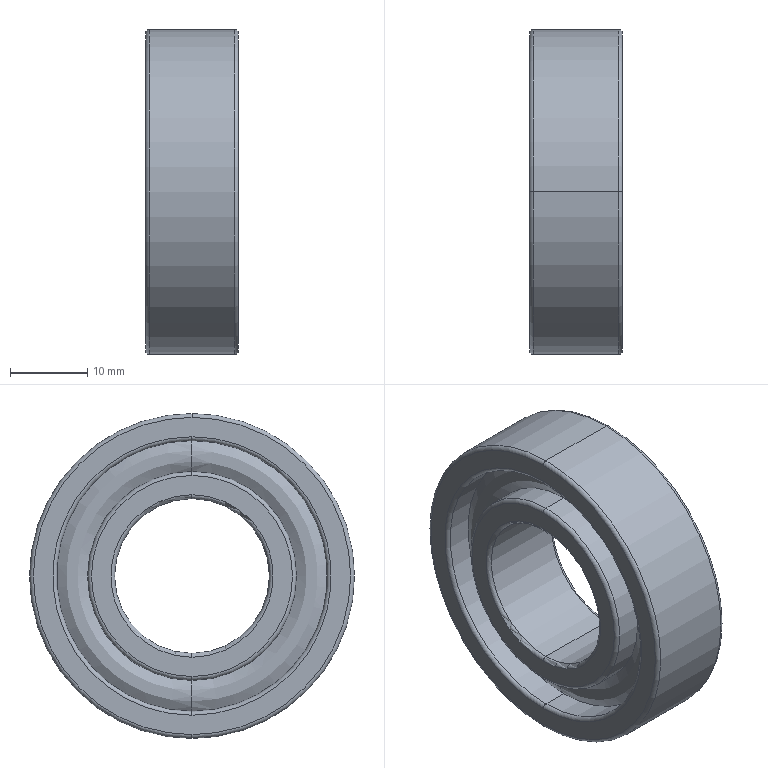Component | SolidWorks | GB-T276  6004RZ-2 | 1 solid | 36 faces | box 12 x 42 x 42 mm | volume 10289 mm3 | torus 20 | cylinder 12 | plane 4 | commonest cylinder face diameters 27 x4 35 x4 42 x2 20 x2 | material '-
build123d program:
from build123d import *

# Parameters (mm, degrees)
FILLET1_R = 0.5


with BuildPart() as part:
    # Sketch1 → Revolve1 (revolve)
    with BuildSketch(Plane.XY, mode=Mode.PRIVATE) as revolve1_sk:
        with BuildLine():
            Line((0, 10), (12, 10))
            Line((12, 10), (12, 13.5))
            Line((12, 13.5), (8.236, 13.5))
            ThreePointArc((8.236, 13.5), (9, 15.5), (8.236, 17.5))
            Line((8.236, 17.5), (12, 17.5))
            Line((12, 17.5), (12, 21))
            Line((12, 21), (0, 21))
            Line((0, 21), (0, 17.5))
            Line((0, 17.5), (3.764, 17.5))
            ThreePointArc((3.764, 17.5), (3, 15.5), (3.764, 13.5))
            Line((3.764, 13.5), (0, 13.5))
            Line((0, 13.5), (0, 10))
        make_face()
    revolve(revolve1_sk.sketch.rotate(Axis((0, 0, 0), (1, 0, 0)), 90), axis=Axis((0, 0, 0), (1, 0, 0)))

    # Fillet1
    fillet1_edges = [part.edges().sort_by_distance(p)[0] for p in [
        (0, 0, -21),
        (12, 0, -21),
        (12, 0, -17.5),
        (12, 0, -13.5),
        (12, 0, -10),
        (0, 0, -10),
        (0, 0, -13.5),
        (0, 0, -17.5),
    ]]
    fillet(fillet1_edges, radius=FILLET1_R)


solid = part.part

# Placed as in the assembly
solid = solid.moved(Location((477, 30, 0), (0, 0, 0)))
STEP:
#1=CARTESIAN_POINT('',(18.78,1.181,-0.5118));
#2=VERTEX_POINT('',#1);
#3=CARTESIAN_POINT('',(18.78,1.181,0.5118));
#4=VERTEX_POINT('',#3);
#5=CARTESIAN_POINT('',(18.78,1.181,-0.));
#6=DIRECTION('',(-1.,-0.,0.));
#7=DIRECTION('',(0.,-0.,1.));
#8=AXIS2_PLACEMENT_3D('',#5,#6,#7);
#9=CIRCLE('',#8,0.5118);
#10=EDGE_CURVE('',#2,#4,#9,.T.);
#11=ORIENTED_EDGE('',*,*,#10,.F.);
#12=CARTESIAN_POINT('',(18.799,1.181,-0.5315));
#13=VERTEX_POINT('',#12);
#14=CARTESIAN_POINT('',(18.799,1.181,-0.5118));
#15=DIRECTION('',(0.,-1.,-0.));
#16=DIRECTION('',(0.,0.,-1.));
#17=AXIS2_PLACEMENT_3D('',#14,#15,#16);
#18=CIRCLE('',#17,0.01969);
#19=EDGE_CURVE('',#2,#13,#18,.T.);
#20=ORIENTED_EDGE('',*,*,#19,.T.);
#21=CARTESIAN_POINT('',(18.799,1.181,0.5315));
#22=VERTEX_POINT('',#21);
#23=CARTESIAN_POINT('',(18.799,1.181,-0.));
#24=DIRECTION('',(1.,0.,-0.));
#25=DIRECTION('',(0.,-0.,1.));
#26=AXIS2_PLACEMENT_3D('',#23,#24,#25);
#27=CIRCLE('',#26,0.5315);
#28=EDGE_CURVE('',#22,#13,#27,.T.);
#29=ORIENTED_EDGE('',*,*,#28,.F.);
#30=CARTESIAN_POINT('',(18.799,1.181,0.5118));
#31=DIRECTION('',(-0.,1.,0.));
#32=DIRECTION('',(0.,0.,1.));
#33=AXIS2_PLACEMENT_3D('',#30,#31,#32);
#34=CIRCLE('',#33,0.01969);
#35=EDGE_CURVE('',#4,#22,#34,.T.);
#36=ORIENTED_EDGE('',*,*,#35,.F.);
#37=EDGE_LOOP('',(#11,#20,#29,#36));
#38=FACE_OUTER_BOUND('',#37,.T.);
#39=CARTESIAN_POINT('',(18.799,1.181,-0.));
#40=DIRECTION('',(1.,0.,-0.));
#41=DIRECTION('',(0.,-0.,1.));
#42=AXIS2_PLACEMENT_3D('',#39,#40,#41);
#43=TOROIDAL_SURFACE('',#42,0.5118,0.01969);
#44=ADVANCED_FACE('',(#38),#43,.T.);
#45=CARTESIAN_POINT('',(18.799,1.181,-0.3937));
#46=VERTEX_POINT('',#45);
#47=CARTESIAN_POINT('',(18.799,1.181,0.3937));
#48=VERTEX_POINT('',#47);
#49=CARTESIAN_POINT('',(18.799,1.181,-0.));
#50=DIRECTION('',(-1.,-0.,0.));
#51=DIRECTION('',(0.,-0.,1.));
#52=AXIS2_PLACEMENT_3D('',#49,#50,#51);
#53=CIRCLE('',#52,0.3937);
#54=EDGE_CURVE('',#46,#48,#53,.T.);
#55=ORIENTED_EDGE('',*,*,#54,.F.);
#56=CARTESIAN_POINT('',(18.78,1.181,-0.4134));
#57=VERTEX_POINT('',#56);
#58=CARTESIAN_POINT('',(18.799,1.181,-0.4134));
#59=DIRECTION('',(0.,-1.,-0.));
#60=DIRECTION('',(0.,0.,-1.));
#61=AXIS2_PLACEMENT_3D('',#58,#59,#60);
#62=CIRCLE('',#61,0.01969);
#63=EDGE_CURVE('',#46,#57,#62,.T.);
#64=ORIENTED_EDGE('',*,*,#63,.T.);
#65=CARTESIAN_POINT('',(18.78,1.181,0.4134));
#66=VERTEX_POINT('',#65);
#67=CARTESIAN_POINT('',(18.78,1.181,-0.));
#68=DIRECTION('',(1.,0.,-0.));
#69=DIRECTION('',(0.,-0.,1.));
#70=AXIS2_PLACEMENT_3D('',#67,#68,#69);
#71=CIRCLE('',#70,0.4134);
#72=EDGE_CURVE('',#66,#57,#71,.T.);
#73=ORIENTED_EDGE('',*,*,#72,.F.);
#74=CARTESIAN_POINT('',(18.799,1.181,0.4134));
#75=DIRECTION('',(-0.,1.,0.));
#76=DIRECTION('',(0.,0.,1.));
#77=AXIS2_PLACEMENT_3D('',#74,#75,#76);
#78=CIRCLE('',#77,0.01969);
#79=EDGE_CURVE('',#48,#66,#78,.T.);
#80=ORIENTED_EDGE('',*,*,#79,.F.);
#81=EDGE_LOOP('',(#55,#64,#73,#80));
#82=FACE_OUTER_BOUND('',#81,.T.);
#83=CARTESIAN_POINT('',(18.799,1.181,-0.));
#84=DIRECTION('',(1.,0.,-0.));
#85=DIRECTION('',(0.,-0.,1.));
#86=AXIS2_PLACEMENT_3D('',#83,#84,#85);
#87=TOROIDAL_SURFACE('',#86,0.4134,0.01969);
#88=ADVANCED_FACE('',(#82),#87,.T.);
#89=CARTESIAN_POINT('',(18.78,1.181,-0.8071));
#90=VERTEX_POINT('',#89);
#91=CARTESIAN_POINT('',(18.78,1.181,0.8071));
#92=VERTEX_POINT('',#91);
#93=CARTESIAN_POINT('',(18.78,1.181,-0.));
#94=DIRECTION('',(-1.,-0.,0.));
#95=DIRECTION('',(0.,-0.,1.));
#96=AXIS2_PLACEMENT_3D('',#93,#94,#95);
#97=CIRCLE('',#96,0.8071);
#98=EDGE_CURVE('',#90,#92,#97,.T.);
#99=ORIENTED_EDGE('',*,*,#98,.F.);
#100=CARTESIAN_POINT('',(18.799,1.181,-0.8268));
#101=VERTEX_POINT('',#100);
#102=CARTESIAN_POINT('',(18.799,1.181,-0.8071));
#103=DIRECTION('',(0.,-1.,-0.));
#104=DIRECTION('',(0.,0.,-1.));
#105=AXIS2_PLACEMENT_3D('',#102,#103,#104);
#106=CIRCLE('',#105,0.01969);
#107=EDGE_CURVE('',#90,#101,#106,.T.);
#108=ORIENTED_EDGE('',*,*,#107,.T.);
#109=CARTESIAN_POINT('',(18.799,1.181,0.8268));
#110=VERTEX_POINT('',#109);
#111=CARTESIAN_POINT('',(18.799,1.181,-0.));
#112=DIRECTION('',(1.,0.,-0.));
#113=DIRECTION('',(0.,-0.,1.));
#114=AXIS2_PLACEMENT_3D('',#111,#112,#113);
#115=CIRCLE('',#114,0.8268);
#116=EDGE_CURVE('',#110,#101,#115,.T.);
#117=ORIENTED_EDGE('',*,*,#116,.F.);
#118=CARTESIAN_POINT('',(18.799,1.181,0.8071));
#119=DIRECTION('',(-0.,1.,0.));
#120=DIRECTION('',(0.,0.,1.));
#121=AXIS2_PLACEMENT_3D('',#118,#119,#120);
#122=CIRCLE('',#121,0.01969);
#123=EDGE_CURVE('',#92,#110,#122,.T.);
#124=ORIENTED_EDGE('',*,*,#123,.F.);
#125=EDGE_LOOP('',(#99,#108,#117,#124));
#126=FACE_OUTER_BOUND('',#125,.T.);
#127=CARTESIAN_POINT('',(18.799,1.181,-0.));
#128=DIRECTION('',(1.,0.,-0.));
#129=DIRECTION('',(0.,-0.,1.));
#130=AXIS2_PLACEMENT_3D('',#127,#128,#129);
#131=TOROIDAL_SURFACE('',#130,0.8071,0.01969);
#132=ADVANCED_FACE('',(#126),#131,.T.);
#133=CARTESIAN_POINT('',(18.799,1.181,-0.689));
#134=VERTEX_POINT('',#133);
#135=CARTESIAN_POINT('',(18.799,1.181,0.689));
#136=VERTEX_POINT('',#135);
#137=CARTESIAN_POINT('',(18.799,1.181,-0.));
#138=DIRECTION('',(-1.,-0.,0.));
#139=DIRECTION('',(0.,-0.,1.));
#140=AXIS2_PLACEMENT_3D('',#137,#138,#139);
#141=CIRCLE('',#140,0.689);
#142=EDGE_CURVE('',#134,#136,#141,.T.);
#143=ORIENTED_EDGE('',*,*,#142,.F.);
#144=CARTESIAN_POINT('',(18.78,1.181,-0.7087));
#145=VERTEX_POINT('',#144);
#146=CARTESIAN_POINT('',(18.799,1.181,-0.7087));
#147=DIRECTION('',(0.,-1.,-0.));
#148=DIRECTION('',(0.,0.,-1.));
#149=AXIS2_PLACEMENT_3D('',#146,#147,#148);
#150=CIRCLE('',#149,0.01969);
#151=EDGE_CURVE('',#134,#145,#150,.T.);
#152=ORIENTED_EDGE('',*,*,#151,.T.);
#153=CARTESIAN_POINT('',(18.78,1.181,0.7087));
#154=VERTEX_POINT('',#153);
#155=CARTESIAN_POINT('',(18.78,1.181,-0.));
#156=DIRECTION('',(1.,0.,-0.));
#157=DIRECTION('',(0.,-0.,1.));
#158=AXIS2_PLACEMENT_3D('',#155,#156,#157);
#159=CIRCLE('',#158,0.7087);
#160=EDGE_CURVE('',#154,#145,#159,.T.);
#161=ORIENTED_EDGE('',*,*,#160,.F.);
#162=CARTESIAN_POINT('',(18.799,1.181,0.7087));
#163=DIRECTION('',(-0.,1.,0.));
#164=DIRECTION('',(0.,0.,1.));
#165=AXIS2_PLACEMENT_3D('',#162,#163,#164);
#166=CIRCLE('',#165,0.01969);
#167=EDGE_CURVE('',#136,#154,#166,.T.);
#168=ORIENTED_EDGE('',*,*,#167,.F.);
#169=EDGE_LOOP('',(#143,#152,#161,#168));
#170=FACE_OUTER_BOUND('',#169,.T.);
#171=CARTESIAN_POINT('',(18.799,1.181,-0.));
#172=DIRECTION('',(1.,0.,-0.));
#173=DIRECTION('',(0.,-0.,1.));
#174=AXIS2_PLACEMENT_3D('',#171,#172,#173);
#175=TOROIDAL_SURFACE('',#174,0.7087,0.01969);
#176=ADVANCED_FACE('',(#170),#175,.T.);
#177=CARTESIAN_POINT('',(19.232,1.181,0.3937));
#178=VERTEX_POINT('',#177);
#179=CARTESIAN_POINT('',(19.232,1.181,-0.3937));
#180=VERTEX_POINT('',#179);
#181=CARTESIAN_POINT('',(19.232,1.181,-0.));
#182=DIRECTION('',(1.,0.,-0.));
#183=DIRECTION('',(0.,0.,-1.));
#184=AXIS2_PLACEMENT_3D('',#181,#182,#183);
#185=CIRCLE('',#184,0.3937);
#186=EDGE_CURVE('',#178,#180,#185,.T.);
#187=ORIENTED_EDGE('',*,*,#186,.F.);
#188=CARTESIAN_POINT('',(19.252,1.181,0.4134));
#189=VERTEX_POINT('',#188);
#190=CARTESIAN_POINT('',(19.232,1.181,0.4134));
#191=DIRECTION('',(0.,-1.,-0.));
#192=DIRECTION('',(0.,0.,-1.));
#193=AXIS2_PLACEMENT_3D('',#190,#191,#192);
#194=CIRCLE('',#193,0.01969);
#195=EDGE_CURVE('',#178,#189,#194,.T.);
#196=ORIENTED_EDGE('',*,*,#195,.T.);
#197=CARTESIAN_POINT('',(19.252,1.181,-0.4134));
#198=VERTEX_POINT('',#197);
#199=CARTESIAN_POINT('',(19.252,1.181,-0.));
#200=DIRECTION('',(-1.,-0.,0.));
#201=DIRECTION('',(0.,0.,-1.));
#202=AXIS2_PLACEMENT_3D('',#199,#200,#201);
#203=CIRCLE('',#202,0.4134);
#204=EDGE_CURVE('',#198,#189,#203,.T.);
#205=ORIENTED_EDGE('',*,*,#204,.F.);
#206=CARTESIAN_POINT('',(19.232,1.181,-0.4134));
#207=DIRECTION('',(-0.,1.,0.));
#208=DIRECTION('',(0.,0.,1.));
#209=AXIS2_PLACEMENT_3D('',#206,#207,#208);
#210=CIRCLE('',#209,0.01969);
#211=EDGE_CURVE('',#180,#198,#210,.T.);
#212=ORIENTED_EDGE('',*,*,#211,.F.);
#213=EDGE_LOOP('',(#187,#196,#205,#212));
#214=FACE_OUTER_BOUND('',#213,.T.);
#215=CARTESIAN_POINT('',(19.232,1.181,-0.));
#216=DIRECTION('',(-1.,-0.,0.));
#217=DIRECTION('',(-0.,0.,-1.));
#218=AXIS2_PLACEMENT_3D('',#215,#216,#217);
#219=TOROIDAL_SURFACE('',#218,0.4134,0.01969);
#220=ADVANCED_FACE('',(#214),#219,.T.);
#221=CARTESIAN_POINT('',(19.252,1.181,0.5118));
#222=VERTEX_POINT('',#221);
#223=CARTESIAN_POINT('',(19.252,1.181,-0.5118));
#224=VERTEX_POINT('',#223);
#225=CARTESIAN_POINT('',(19.252,1.181,-0.));
#226=DIRECTION('',(1.,0.,-0.));
#227=DIRECTION('',(0.,0.,-1.));
#228=AXIS2_PLACEMENT_3D('',#225,#226,#227);
#229=CIRCLE('',#228,0.5118);
#230=EDGE_CURVE('',#222,#224,#229,.T.);
#231=ORIENTED_EDGE('',*,*,#230,.F.);
#232=CARTESIAN_POINT('',(19.232,1.181,0.5315));
#233=VERTEX_POINT('',#232);
#234=CARTESIAN_POINT('',(19.232,1.181,0.5118));
#235=DIRECTION('',(0.,-1.,-0.));
#236=DIRECTION('',(0.,0.,-1.));
#237=AXIS2_PLACEMENT_3D('',#234,#235,#236);
#238=CIRCLE('',#237,0.01969);
#239=EDGE_CURVE('',#222,#233,#238,.T.);
#240=ORIENTED_EDGE('',*,*,#239,.T.);
#241=CARTESIAN_POINT('',(19.232,1.181,-0.5315));
#242=VERTEX_POINT('',#241);
#243=CARTESIAN_POINT('',(19.232,1.181,-0.));
#244=DIRECTION('',(-1.,-0.,0.));
#245=DIRECTION('',(0.,0.,-1.));
#246=AXIS2_PLACEMENT_3D('',#243,#244,#245);
#247=CIRCLE('',#246,0.5315);
#248=EDGE_CURVE('',#242,#233,#247,.T.);
#249=ORIENTED_EDGE('',*,*,#248,.F.);
#250=CARTESIAN_POINT('',(19.232,1.181,-0.5118));
#251=DIRECTION('',(-0.,1.,0.));
#252=DIRECTION('',(0.,0.,1.));
#253=AXIS2_PLACEMENT_3D('',#250,#251,#252);
#254=CIRCLE('',#253,0.01969);
#255=EDGE_CURVE('',#224,#242,#254,.T.);
#256=ORIENTED_EDGE('',*,*,#255,.F.);
#257=EDGE_LOOP('',(#231,#240,#249,#256));
#258=FACE_OUTER_BOUND('',#257,.T.);
#259=CARTESIAN_POINT('',(19.232,1.181,-0.));
#260=DIRECTION('',(-1.,-0.,0.));
#261=DIRECTION('',(-0.,0.,-1.));
#262=AXIS2_PLACEMENT_3D('',#259,#260,#261);
#263=TOROIDAL_SURFACE('',#262,0.5118,0.01969);
#264=ADVANCED_FACE('',(#258),#263,.T.);
#265=CARTESIAN_POINT('',(19.232,1.181,0.689));
#266=VERTEX_POINT('',#265);
#267=CARTESIAN_POINT('',(19.232,1.181,-0.689));
#268=VERTEX_POINT('',#267);
#269=CARTESIAN_POINT('',(19.232,1.181,-0.));
#270=DIRECTION('',(1.,0.,-0.));
#271=DIRECTION('',(0.,0.,-1.));
#272=AXIS2_PLACEMENT_3D('',#269,#270,#271);
#273=CIRCLE('',#272,0.689);
#274=EDGE_CURVE('',#266,#268,#273,.T.);
#275=ORIENTED_EDGE('',*,*,#274,.F.);
#276=CARTESIAN_POINT('',(19.252,1.181,0.7087));
#277=VERTEX_POINT('',#276);
#278=CARTESIAN_POINT('',(19.232,1.181,0.7087));
#279=DIRECTION('',(0.,-1.,-0.));
#280=DIRECTION('',(0.,0.,-1.));
#281=AXIS2_PLACEMENT_3D('',#278,#279,#280);
#282=CIRCLE('',#281,0.01969);
#283=EDGE_CURVE('',#266,#277,#282,.T.);
#284=ORIENTED_EDGE('',*,*,#283,.T.);
#285=CARTESIAN_POINT('',(19.252,1.181,-0.7087));
#286=VERTEX_POINT('',#285);
#287=CARTESIAN_POINT('',(19.252,1.181,-0.));
#288=DIRECTION('',(-1.,-0.,0.));
#289=DIRECTION('',(0.,0.,-1.));
#290=AXIS2_PLACEMENT_3D('',#287,#288,#289);
#291=CIRCLE('',#290,0.7087);
#292=EDGE_CURVE('',#286,#277,#291,.T.);
#293=ORIENTED_EDGE('',*,*,#292,.F.);
#294=CARTESIAN_POINT('',(19.232,1.181,-0.7087));
#295=DIRECTION('',(-0.,1.,0.));
#296=DIRECTION('',(0.,0.,1.));
#297=AXIS2_PLACEMENT_3D('',#294,#295,#296);
#298=CIRCLE('',#297,0.01969);
#299=EDGE_CURVE('',#268,#286,#298,.T.);
#300=ORIENTED_EDGE('',*,*,#299,.F.);
#301=EDGE_LOOP('',(#275,#284,#293,#300));
#302=FACE_OUTER_BOUND('',#301,.T.);
#303=CARTESIAN_POINT('',(19.232,1.181,-0.));
#304=DIRECTION('',(-1.,-0.,0.));
#305=DIRECTION('',(-0.,0.,-1.));
#306=AXIS2_PLACEMENT_3D('',#303,#304,#305);
#307=TOROIDAL_SURFACE('',#306,0.7087,0.01969);
#308=ADVANCED_FACE('',(#302),#307,.T.);
#309=CARTESIAN_POINT('',(19.252,1.181,0.8071));
#310=VERTEX_POINT('',#309);
#311=CARTESIAN_POINT('',(19.252,1.181,-0.8071));
#312=VERTEX_POINT('',#311);
#313=CARTESIAN_POINT('',(19.252,1.181,-0.));
#314=DIRECTION('',(1.,0.,-0.));
#315=DIRECTION('',(0.,0.,-1.));
#316=AXIS2_PLACEMENT_3D('',#313,#314,#315);
#317=CIRCLE('',#316,0.8071);
#318=EDGE_CURVE('',#310,#312,#317,.T.);
#319=ORIENTED_EDGE('',*,*,#318,.F.);
#320=CARTESIAN_POINT('',(19.232,1.181,0.8268));
#321=VERTEX_POINT('',#320);
#322=CARTESIAN_POINT('',(19.232,1.181,0.8071));
#323=DIRECTION('',(0.,-1.,-0.));
#324=DIRECTION('',(0.,0.,-1.));
#325=AXIS2_PLACEMENT_3D('',#322,#323,#324);
#326=CIRCLE('',#325,0.01969);
#327=EDGE_CURVE('',#310,#321,#326,.T.);
#328=ORIENTED_EDGE('',*,*,#327,.T.);
#329=CARTESIAN_POINT('',(19.232,1.181,-0.8268));
#330=VERTEX_POINT('',#329);
#331=CARTESIAN_POINT('',(19.232,1.181,-0.));
#332=DIRECTION('',(-1.,-0.,0.));
#333=DIRECTION('',(0.,0.,-1.));
#334=AXIS2_PLACEMENT_3D('',#331,#332,#333);
#335=CIRCLE('',#334,0.8268);
#336=EDGE_CURVE('',#330,#321,#335,.T.);
#337=ORIENTED_EDGE('',*,*,#336,.F.);
#338=CARTESIAN_POINT('',(19.232,1.181,-0.8071));
#339=DIRECTION('',(-0.,1.,0.));
#340=DIRECTION('',(0.,0.,1.));
#341=AXIS2_PLACEMENT_3D('',#338,#339,#340);
#342=CIRCLE('',#341,0.01969);
#343=EDGE_CURVE('',#312,#330,#342,.T.);
#344=ORIENTED_EDGE('',*,*,#343,.F.);
#345=EDGE_LOOP('',(#319,#328,#337,#344));
#346=FACE_OUTER_BOUND('',#345,.T.);
#347=CARTESIAN_POINT('',(19.232,1.181,-0.));
#348=DIRECTION('',(-1.,-0.,0.));
#349=DIRECTION('',(-0.,0.,-1.));
#350=AXIS2_PLACEMENT_3D('',#347,#348,#349);
#351=TOROIDAL_SURFACE('',#350,0.8071,0.01969);
#352=ADVANCED_FACE('',(#346),#351,.T.);
#353=CARTESIAN_POINT('',(19.104,1.181,0.5315));
#354=VERTEX_POINT('',#353);
#355=CARTESIAN_POINT('',(19.104,1.181,-0.5315));
#356=VERTEX_POINT('',#355);
#357=CARTESIAN_POINT('',(19.104,1.181,-0.));
#358=DIRECTION('',(1.,0.,-0.));
#359=DIRECTION('',(0.,-0.,1.));
#360=AXIS2_PLACEMENT_3D('',#357,#358,#359);
#361=CIRCLE('',#360,0.5315);
#362=EDGE_CURVE('',#354,#356,#361,.T.);
#363=ORIENTED_EDGE('',*,*,#362,.T.);
#364=CARTESIAN_POINT('',(19.252,1.181,-0.5315));
#365=DIRECTION('',(1.,0.,-0.));
#366=VECTOR('',#365,39.37);
#367=LINE('',#364,#366);
#368=EDGE_CURVE('',#356,#242,#367,.T.);
#369=ORIENTED_EDGE('',*,*,#368,.T.);
#370=ORIENTED_EDGE('',*,*,#248,.T.);
#371=CARTESIAN_POINT('',(19.252,1.181,0.5315));
#372=DIRECTION('',(1.,0.,-0.));
#373=VECTOR('',#372,39.37);
#374=LINE('',#371,#373);
#375=EDGE_CURVE('',#354,#233,#374,.T.);
#376=ORIENTED_EDGE('',*,*,#375,.F.);
#377=EDGE_LOOP('',(#363,#369,#370,#376));
#378=FACE_OUTER_BOUND('',#377,.T.);
#379=CARTESIAN_POINT('',(19.252,1.181,-0.));
#380=DIRECTION('',(1.,0.,-0.));
#381=DIRECTION('',(0.,-0.,1.));
#382=AXIS2_PLACEMENT_3D('',#379,#380,#381);
#383=CYLINDRICAL_SURFACE('',#382,0.5315);
#384=ADVANCED_FACE('',(#378),#383,.T.);
#385=CARTESIAN_POINT('',(19.104,1.181,0.689));
#386=VERTEX_POINT('',#385);
#387=CARTESIAN_POINT('',(19.104,1.181,-0.689));
#388=VERTEX_POINT('',#387);
#389=CARTESIAN_POINT('',(19.104,1.181,-0.));
#390=DIRECTION('',(1.,0.,-0.));
#391=DIRECTION('',(0.,-0.,1.));
#392=AXIS2_PLACEMENT_3D('',#389,#390,#391);
#393=CIRCLE('',#392,0.689);
#394=EDGE_CURVE('',#386,#388,#393,.T.);
#395=ORIENTED_EDGE('',*,*,#394,.T.);
#396=CARTESIAN_POINT('',(19.016,1.181,-0.6102));
#397=DIRECTION('',(0.,-1.,-0.));
#398=DIRECTION('',(0.,0.,-1.));
#399=AXIS2_PLACEMENT_3D('',#396,#397,#398);
#400=CIRCLE('',#399,0.1181);
#401=EDGE_CURVE('',#388,#356,#400,.T.);
#402=ORIENTED_EDGE('',*,*,#401,.T.);
#403=ORIENTED_EDGE('',*,*,#362,.F.);
#404=CARTESIAN_POINT('',(19.016,1.181,0.6102));
#405=DIRECTION('',(-0.,1.,0.));
#406=DIRECTION('',(0.,0.,1.));
#407=AXIS2_PLACEMENT_3D('',#404,#405,#406);
#408=CIRCLE('',#407,0.1181);
#409=EDGE_CURVE('',#386,#354,#408,.T.);
#410=ORIENTED_EDGE('',*,*,#409,.F.);
#411=EDGE_LOOP('',(#395,#402,#403,#410));
#412=FACE_OUTER_BOUND('',#411,.T.);
#413=CARTESIAN_POINT('',(19.016,1.181,-0.));
#414=DIRECTION('',(1.,0.,-0.));
#415=DIRECTION('',(0.,-0.,1.));
#416=AXIS2_PLACEMENT_3D('',#413,#414,#415);
#417=TOROIDAL_SURFACE('',#416,0.6102,0.1181);
#418=ADVANCED_FACE('',(#412),#417,.T.);
#419=CARTESIAN_POINT('',(19.104,1.181,-0.));
#420=DIRECTION('',(1.,0.,-0.));
#421=DIRECTION('',(0.,-0.,1.));
#422=AXIS2_PLACEMENT_3D('',#419,#420,#421);
#423=CIRCLE('',#422,0.689);
#424=EDGE_CURVE('',#388,#386,#423,.T.);
#425=ORIENTED_EDGE('',*,*,#424,.F.);
#426=CARTESIAN_POINT('',(19.252,1.181,-0.689));
#427=DIRECTION('',(1.,0.,-0.));
#428=VECTOR('',#427,39.37);
#429=LINE('',#426,#428);
#430=EDGE_CURVE('',#388,#268,#429,.T.);
#431=ORIENTED_EDGE('',*,*,#430,.T.);
#432=CARTESIAN_POINT('',(19.232,1.181,-0.));
#433=DIRECTION('',(1.,0.,-0.));
#434=DIRECTION('',(0.,0.,-1.));
#435=AXIS2_PLACEMENT_3D('',#432,#433,#434);
#436=CIRCLE('',#435,0.689);
#437=EDGE_CURVE('',#268,#266,#436,.T.);
#438=ORIENTED_EDGE('',*,*,#437,.T.);
#439=CARTESIAN_POINT('',(19.252,1.181,0.689));
#440=DIRECTION('',(1.,0.,-0.));
#441=VECTOR('',#440,39.37);
#442=LINE('',#439,#441);
#443=EDGE_CURVE('',#386,#266,#442,.T.);
#444=ORIENTED_EDGE('',*,*,#443,.F.);
#445=EDGE_LOOP('',(#425,#431,#438,#444));
#446=FACE_OUTER_BOUND('',#445,.T.);
#447=CARTESIAN_POINT('',(19.252,1.181,-0.));
#448=DIRECTION('',(1.,0.,-0.));
#449=DIRECTION('',(0.,-0.,1.));
#450=AXIS2_PLACEMENT_3D('',#447,#448,#449);
#451=CYLINDRICAL_SURFACE('',#450,0.689);
#452=ADVANCED_FACE('',(#446),#451,.F.);
#453=ORIENTED_EDGE('',*,*,#116,.T.);
#454=CARTESIAN_POINT('',(19.252,1.181,-0.8268));
#455=DIRECTION('',(1.,0.,-0.));
#456=VECTOR('',#455,39.37);
#457=LINE('',#454,#456);
#458=EDGE_CURVE('',#101,#330,#457,.T.);
#459=ORIENTED_EDGE('',*,*,#458,.T.);
#460=ORIENTED_EDGE('',*,*,#336,.T.);
#461=CARTESIAN_POINT('',(19.252,1.181,0.8268));
#462=DIRECTION('',(1.,0.,-0.));
#463=VECTOR('',#462,39.37);
#464=LINE('',#461,#463);
#465=EDGE_CURVE('',#110,#321,#464,.T.);
#466=ORIENTED_EDGE('',*,*,#465,.F.);
#467=EDGE_LOOP('',(#453,#459,#460,#466));
#468=FACE_OUTER_BOUND('',#467,.T.);
#469=CARTESIAN_POINT('',(19.252,1.181,-0.));
#470=DIRECTION('',(1.,0.,-0.));
#471=DIRECTION('',(0.,-0.,1.));
#472=AXIS2_PLACEMENT_3D('',#469,#470,#471);
#473=CYLINDRICAL_SURFACE('',#472,0.8268);
#474=ADVANCED_FACE('',(#468),#473,.T.);
#475=CARTESIAN_POINT('',(18.799,1.181,-0.));
#476=DIRECTION('',(-1.,-0.,0.));
#477=DIRECTION('',(0.,-0.,1.));
#478=AXIS2_PLACEMENT_3D('',#475,#476,#477);
#479=CIRCLE('',#478,0.689);
#480=EDGE_CURVE('',#136,#134,#479,.T.);
#481=ORIENTED_EDGE('',*,*,#480,.T.);
#482=CARTESIAN_POINT('',(18.928,1.181,-0.689));
#483=VERTEX_POINT('',#482);
#484=CARTESIAN_POINT('',(19.252,1.181,-0.689));
#485=DIRECTION('',(1.,0.,-0.));
#486=VECTOR('',#485,39.37);
#487=LINE('',#484,#486);
#488=EDGE_CURVE('',#134,#483,#487,.T.);
#489=ORIENTED_EDGE('',*,*,#488,.T.);
#490=CARTESIAN_POINT('',(18.928,1.181,0.689));
#491=VERTEX_POINT('',#490);
#492=CARTESIAN_POINT('',(18.928,1.181,-0.));
#493=DIRECTION('',(1.,0.,-0.));
#494=DIRECTION('',(0.,-0.,1.));
#495=AXIS2_PLACEMENT_3D('',#492,#493,#494);
#496=CIRCLE('',#495,0.689);
#497=EDGE_CURVE('',#483,#491,#496,.T.);
#498=ORIENTED_EDGE('',*,*,#497,.T.);
#499=CARTESIAN_POINT('',(19.252,1.181,0.689));
#500=DIRECTION('',(1.,0.,-0.));
#501=VECTOR('',#500,39.37);
#502=LINE('',#499,#501);
#503=EDGE_CURVE('',#136,#491,#502,.T.);
#504=ORIENTED_EDGE('',*,*,#503,.F.);
#505=EDGE_LOOP('',(#481,#489,#498,#504));
#506=FACE_OUTER_BOUND('',#505,.T.);
#507=CARTESIAN_POINT('',(19.252,1.181,-0.));
#508=DIRECTION('',(1.,0.,-0.));
#509=DIRECTION('',(0.,-0.,1.));
#510=AXIS2_PLACEMENT_3D('',#507,#508,#509);
#511=CYLINDRICAL_SURFACE('',#510,0.689);
#512=ADVANCED_FACE('',(#506),#511,.F.);
#513=CARTESIAN_POINT('',(18.928,1.181,0.5315));
#514=VERTEX_POINT('',#513);
#515=CARTESIAN_POINT('',(18.928,1.181,-0.5315));
#516=VERTEX_POINT('',#515);
#517=CARTESIAN_POINT('',(18.928,1.181,-0.));
#518=DIRECTION('',(1.,0.,-0.));
#519=DIRECTION('',(0.,-0.,1.));
#520=AXIS2_PLACEMENT_3D('',#517,#518,#519);
#521=CIRCLE('',#520,0.5315);
#522=EDGE_CURVE('',#514,#516,#521,.T.);
#523=ORIENTED_EDGE('',*,*,#522,.T.);
#524=CARTESIAN_POINT('',(19.016,1.181,-0.6102));
#525=DIRECTION('',(0.,-1.,-0.));
#526=DIRECTION('',(0.,0.,-1.));
#527=AXIS2_PLACEMENT_3D('',#524,#525,#526);
#528=CIRCLE('',#527,0.1181);
#529=EDGE_CURVE('',#516,#483,#528,.T.);
#530=ORIENTED_EDGE('',*,*,#529,.T.);
#531=CARTESIAN_POINT('',(18.928,1.181,-0.));
#532=DIRECTION('',(1.,0.,-0.));
#533=DIRECTION('',(0.,-0.,1.));
#534=AXIS2_PLACEMENT_3D('',#531,#532,#533);
#535=CIRCLE('',#534,0.689);
#536=EDGE_CURVE('',#491,#483,#535,.T.);
#537=ORIENTED_EDGE('',*,*,#536,.F.);
#538=CARTESIAN_POINT('',(19.016,1.181,0.6102));
#539=DIRECTION('',(-0.,1.,0.));
#540=DIRECTION('',(0.,0.,1.));
#541=AXIS2_PLACEMENT_3D('',#538,#539,#540);
#542=CIRCLE('',#541,0.1181);
#543=EDGE_CURVE('',#514,#491,#542,.T.);
#544=ORIENTED_EDGE('',*,*,#543,.F.);
#545=EDGE_LOOP('',(#523,#530,#537,#544));
#546=FACE_OUTER_BOUND('',#545,.T.);
#547=CARTESIAN_POINT('',(19.016,1.181,-0.));
#548=DIRECTION('',(1.,0.,-0.));
#549=DIRECTION('',(0.,-0.,1.));
#550=AXIS2_PLACEMENT_3D('',#547,#548,#549);
#551=TOROIDAL_SURFACE('',#550,0.6102,0.1181);
#552=ADVANCED_FACE('',(#546),#551,.T.);
#553=ORIENTED_EDGE('',*,*,#28,.T.);
#554=CARTESIAN_POINT('',(19.252,1.181,-0.5315));
#555=DIRECTION('',(1.,0.,-0.));
#556=VECTOR('',#555,39.37);
#557=LINE('',#554,#556);
#558=EDGE_CURVE('',#13,#516,#557,.T.);
#559=ORIENTED_EDGE('',*,*,#558,.T.);
#560=ORIENTED_EDGE('',*,*,#522,.F.);
#561=CARTESIAN_POINT('',(19.252,1.181,0.5315));
#562=DIRECTION('',(1.,0.,-0.));
#563=VECTOR('',#562,39.37);
#564=LINE('',#561,#563);
#565=EDGE_CURVE('',#22,#514,#564,.T.);
#566=ORIENTED_EDGE('',*,*,#565,.F.);
#567=EDGE_LOOP('',(#553,#559,#560,#566));
#568=FACE_OUTER_BOUND('',#567,.T.);
#569=CARTESIAN_POINT('',(19.252,1.181,-0.));
#570=DIRECTION('',(1.,0.,-0.));
#571=DIRECTION('',(0.,-0.,1.));
#572=AXIS2_PLACEMENT_3D('',#569,#570,#571);
#573=CYLINDRICAL_SURFACE('',#572,0.5315);
#574=ADVANCED_FACE('',(#568),#573,.T.);
#575=CARTESIAN_POINT('',(18.799,1.181,-0.));
#576=DIRECTION('',(-1.,-0.,0.));
#577=DIRECTION('',(0.,-0.,1.));
#578=AXIS2_PLACEMENT_3D('',#575,#576,#577);
#579=CIRCLE('',#578,0.3937);
#580=EDGE_CURVE('',#48,#46,#579,.T.);
#581=ORIENTED_EDGE('',*,*,#580,.T.);
#582=CARTESIAN_POINT('',(19.252,1.181,-0.3937));
#583=DIRECTION('',(1.,0.,-0.));
#584=VECTOR('',#583,39.37);
#585=LINE('',#582,#584);
#586=EDGE_CURVE('',#46,#180,#585,.T.);
#587=ORIENTED_EDGE('',*,*,#586,.T.);
#588=CARTESIAN_POINT('',(19.232,1.181,-0.));
#589=DIRECTION('',(1.,0.,-0.));
#590=DIRECTION('',(0.,0.,-1.));
#591=AXIS2_PLACEMENT_3D('',#588,#589,#590);
#592=CIRCLE('',#591,0.3937);
#593=EDGE_CURVE('',#180,#178,#592,.T.);
#594=ORIENTED_EDGE('',*,*,#593,.T.);
#595=CARTESIAN_POINT('',(19.252,1.181,0.3937));
#596=DIRECTION('',(1.,0.,-0.));
#597=VECTOR('',#596,39.37);
#598=LINE('',#595,#597);
#599=EDGE_CURVE('',#48,#178,#598,.T.);
#600=ORIENTED_EDGE('',*,*,#599,.F.);
#601=EDGE_LOOP('',(#581,#587,#594,#600));
#602=FACE_OUTER_BOUND('',#601,.T.);
#603=CARTESIAN_POINT('',(19.252,1.181,-0.));
#604=DIRECTION('',(1.,0.,-0.));
#605=DIRECTION('',(0.,-0.,1.));
#606=AXIS2_PLACEMENT_3D('',#603,#604,#605);
#607=CYLINDRICAL_SURFACE('',#606,0.3937);
#608=ADVANCED_FACE('',(#602),#607,.F.);
#609=CARTESIAN_POINT('',(19.252,1.181,-0.));
#610=DIRECTION('',(1.,0.,-0.));
#611=DIRECTION('',(0.,0.,-1.));
#612=AXIS2_PLACEMENT_3D('',#609,#610,#611);
#613=CIRCLE('',#612,0.5118);
#614=EDGE_CURVE('',#224,#222,#613,.T.);
#615=ORIENTED_EDGE('',*,*,#614,.T.);
#616=ORIENTED_EDGE('',*,*,#230,.T.);
#617=EDGE_LOOP('',(#615,#616));
#618=FACE_OUTER_BOUND('',#617,.T.);
#619=ORIENTED_EDGE('',*,*,#204,.T.);
#620=CARTESIAN_POINT('',(19.252,1.181,-0.));
#621=DIRECTION('',(-1.,-0.,0.));
#622=DIRECTION('',(0.,0.,-1.));
#623=AXIS2_PLACEMENT_3D('',#620,#621,#622);
#624=CIRCLE('',#623,0.4134);
#625=EDGE_CURVE('',#189,#198,#624,.T.);
#626=ORIENTED_EDGE('',*,*,#625,.T.);
#627=EDGE_LOOP('',(#619,#626));
#628=FACE_BOUND('',#627,.T.);
#629=CARTESIAN_POINT('',(19.252,0.7874,-0.));
#630=DIRECTION('',(-1.,-0.,0.));
#631=DIRECTION('',(-0.,0.,-1.));
#632=AXIS2_PLACEMENT_3D('',#629,#630,#631);
#633=PLANE('',#632);
#634=ADVANCED_FACE('',(#618,#628),#633,.F.);
#635=ORIENTED_EDGE('',*,*,#586,.F.);
#636=ORIENTED_EDGE('',*,*,#54,.T.);
#637=ORIENTED_EDGE('',*,*,#599,.T.);
#638=ORIENTED_EDGE('',*,*,#186,.T.);
#639=EDGE_LOOP('',(#635,#636,#637,#638));
#640=FACE_OUTER_BOUND('',#639,.T.);
#641=CARTESIAN_POINT('',(19.252,1.181,-0.));
#642=DIRECTION('',(1.,0.,-0.));
#643=DIRECTION('',(0.,-0.,1.));
#644=AXIS2_PLACEMENT_3D('',#641,#642,#643);
#645=CYLINDRICAL_SURFACE('',#644,0.3937);
#646=ADVANCED_FACE('',(#640),#645,.F.);
#647=ORIENTED_EDGE('',*,*,#72,.T.);
#648=CARTESIAN_POINT('',(18.78,1.181,-0.));
#649=DIRECTION('',(1.,0.,-0.));
#650=DIRECTION('',(0.,-0.,1.));
#651=AXIS2_PLACEMENT_3D('',#648,#649,#650);
#652=CIRCLE('',#651,0.4134);
#653=EDGE_CURVE('',#57,#66,#652,.T.);
#654=ORIENTED_EDGE('',*,*,#653,.T.);
#655=EDGE_LOOP('',(#647,#654));
#656=FACE_BOUND('',#655,.T.);
#657=CARTESIAN_POINT('',(18.78,1.181,-0.));
#658=DIRECTION('',(-1.,-0.,0.));
#659=DIRECTION('',(0.,-0.,1.));
#660=AXIS2_PLACEMENT_3D('',#657,#658,#659);
#661=CIRCLE('',#660,0.5118);
#662=EDGE_CURVE('',#4,#2,#661,.T.);
#663=ORIENTED_EDGE('',*,*,#662,.T.);
#664=ORIENTED_EDGE('',*,*,#10,.T.);
#665=EDGE_LOOP('',(#663,#664));
#666=FACE_OUTER_BOUND('',#665,.T.);
#667=CARTESIAN_POINT('',(18.78,0.7874,-0.));
#668=DIRECTION('',(1.,0.,-0.));
#669=DIRECTION('',(0.,-0.,1.));
#670=AXIS2_PLACEMENT_3D('',#667,#668,#669);
#671=PLANE('',#670);
#672=ADVANCED_FACE('',(#656,#666),#671,.F.);
#673=ORIENTED_EDGE('',*,*,#558,.F.);
#674=CARTESIAN_POINT('',(18.799,1.181,-0.));
#675=DIRECTION('',(1.,0.,-0.));
#676=DIRECTION('',(0.,-0.,1.));
#677=AXIS2_PLACEMENT_3D('',#674,#675,#676);
#678=CIRCLE('',#677,0.5315);
#679=EDGE_CURVE('',#13,#22,#678,.T.);
#680=ORIENTED_EDGE('',*,*,#679,.T.);
#681=ORIENTED_EDGE('',*,*,#565,.T.);
#682=CARTESIAN_POINT('',(18.928,1.181,-0.));
#683=DIRECTION('',(1.,0.,-0.));
#684=DIRECTION('',(0.,-0.,1.));
#685=AXIS2_PLACEMENT_3D('',#682,#683,#684);
#686=CIRCLE('',#685,0.5315);
#687=EDGE_CURVE('',#516,#514,#686,.T.);
#688=ORIENTED_EDGE('',*,*,#687,.F.);
#689=EDGE_LOOP('',(#673,#680,#681,#688));
#690=FACE_OUTER_BOUND('',#689,.T.);
#691=CARTESIAN_POINT('',(19.252,1.181,-0.));
#692=DIRECTION('',(1.,0.,-0.));
#693=DIRECTION('',(0.,-0.,1.));
#694=AXIS2_PLACEMENT_3D('',#691,#692,#693);
#695=CYLINDRICAL_SURFACE('',#694,0.5315);
#696=ADVANCED_FACE('',(#690),#695,.T.);
#697=ORIENTED_EDGE('',*,*,#529,.F.);
#698=ORIENTED_EDGE('',*,*,#687,.T.);
#699=ORIENTED_EDGE('',*,*,#543,.T.);
#700=ORIENTED_EDGE('',*,*,#497,.F.);
#701=EDGE_LOOP('',(#697,#698,#699,#700));
#702=FACE_OUTER_BOUND('',#701,.T.);
#703=CARTESIAN_POINT('',(19.016,1.181,-0.));
#704=DIRECTION('',(1.,0.,-0.));
#705=DIRECTION('',(0.,-0.,1.));
#706=AXIS2_PLACEMENT_3D('',#703,#704,#705);
#707=TOROIDAL_SURFACE('',#706,0.6102,0.1181);
#708=ADVANCED_FACE('',(#702),#707,.T.);
#709=ORIENTED_EDGE('',*,*,#488,.F.);
#710=ORIENTED_EDGE('',*,*,#142,.T.);
#711=ORIENTED_EDGE('',*,*,#503,.T.);
#712=ORIENTED_EDGE('',*,*,#536,.T.);
#713=EDGE_LOOP('',(#709,#710,#711,#712));
#714=FACE_OUTER_BOUND('',#713,.T.);
#715=CARTESIAN_POINT('',(19.252,1.181,-0.));
#716=DIRECTION('',(1.,0.,-0.));
#717=DIRECTION('',(0.,-0.,1.));
#718=AXIS2_PLACEMENT_3D('',#715,#716,#717);
#719=CYLINDRICAL_SURFACE('',#718,0.689);
#720=ADVANCED_FACE('',(#714),#719,.F.);
#721=ORIENTED_EDGE('',*,*,#160,.T.);
#722=CARTESIAN_POINT('',(18.78,1.181,-0.));
#723=DIRECTION('',(1.,0.,-0.));
#724=DIRECTION('',(0.,-0.,1.));
#725=AXIS2_PLACEMENT_3D('',#722,#723,#724);
#726=CIRCLE('',#725,0.7087);
#727=EDGE_CURVE('',#145,#154,#726,.T.);
#728=ORIENTED_EDGE('',*,*,#727,.T.);
#729=EDGE_LOOP('',(#721,#728));
#730=FACE_BOUND('',#729,.T.);
#731=CARTESIAN_POINT('',(18.78,1.181,-0.));
#732=DIRECTION('',(-1.,-0.,0.));
#733=DIRECTION('',(0.,-0.,1.));
#734=AXIS2_PLACEMENT_3D('',#731,#732,#733);
#735=CIRCLE('',#734,0.8071);
#736=EDGE_CURVE('',#92,#90,#735,.T.);
#737=ORIENTED_EDGE('',*,*,#736,.T.);
#738=ORIENTED_EDGE('',*,*,#98,.T.);
#739=EDGE_LOOP('',(#737,#738));
#740=FACE_OUTER_BOUND('',#739,.T.);
#741=CARTESIAN_POINT('',(18.78,0.4921,-0.));
#742=DIRECTION('',(1.,0.,-0.));
#743=DIRECTION('',(0.,-0.,1.));
#744=AXIS2_PLACEMENT_3D('',#741,#742,#743);
#745=PLANE('',#744);
#746=ADVANCED_FACE('',(#730,#740),#745,.F.);
#747=ORIENTED_EDGE('',*,*,#458,.F.);
#748=CARTESIAN_POINT('',(18.799,1.181,-0.));
#749=DIRECTION('',(1.,0.,-0.));
#750=DIRECTION('',(0.,-0.,1.));
#751=AXIS2_PLACEMENT_3D('',#748,#749,#750);
#752=CIRCLE('',#751,0.8268);
#753=EDGE_CURVE('',#101,#110,#752,.T.);
#754=ORIENTED_EDGE('',*,*,#753,.T.);
#755=ORIENTED_EDGE('',*,*,#465,.T.);
#756=CARTESIAN_POINT('',(19.232,1.181,-0.));
#757=DIRECTION('',(-1.,-0.,0.));
#758=DIRECTION('',(0.,0.,-1.));
#759=AXIS2_PLACEMENT_3D('',#756,#757,#758);
#760=CIRCLE('',#759,0.8268);
#761=EDGE_CURVE('',#321,#330,#760,.T.);
#762=ORIENTED_EDGE('',*,*,#761,.T.);
#763=EDGE_LOOP('',(#747,#754,#755,#762));
#764=FACE_OUTER_BOUND('',#763,.T.);
#765=CARTESIAN_POINT('',(19.252,1.181,-0.));
#766=DIRECTION('',(1.,0.,-0.));
#767=DIRECTION('',(0.,-0.,1.));
#768=AXIS2_PLACEMENT_3D('',#765,#766,#767);
#769=CYLINDRICAL_SURFACE('',#768,0.8268);
#770=ADVANCED_FACE('',(#764),#769,.T.);
#771=CARTESIAN_POINT('',(19.252,1.181,-0.));
#772=DIRECTION('',(1.,0.,-0.));
#773=DIRECTION('',(0.,0.,-1.));
#774=AXIS2_PLACEMENT_3D('',#771,#772,#773);
#775=CIRCLE('',#774,0.8071);
#776=EDGE_CURVE('',#312,#310,#775,.T.);
#777=ORIENTED_EDGE('',*,*,#776,.T.);
#778=ORIENTED_EDGE('',*,*,#318,.T.);
#779=EDGE_LOOP('',(#777,#778));
#780=FACE_OUTER_BOUND('',#779,.T.);
#781=ORIENTED_EDGE('',*,*,#292,.T.);
#782=CARTESIAN_POINT('',(19.252,1.181,-0.));
#783=DIRECTION('',(-1.,-0.,0.));
#784=DIRECTION('',(0.,0.,-1.));
#785=AXIS2_PLACEMENT_3D('',#782,#783,#784);
#786=CIRCLE('',#785,0.7087);
#787=EDGE_CURVE('',#277,#286,#786,.T.);
#788=ORIENTED_EDGE('',*,*,#787,.T.);
#789=EDGE_LOOP('',(#781,#788));
#790=FACE_BOUND('',#789,.T.);
#791=CARTESIAN_POINT('',(19.252,0.4921,-0.));
#792=DIRECTION('',(-1.,-0.,0.));
#793=DIRECTION('',(-0.,0.,-1.));
#794=AXIS2_PLACEMENT_3D('',#791,#792,#793);
#795=PLANE('',#794);
#796=ADVANCED_FACE('',(#780,#790),#795,.F.);
#797=ORIENTED_EDGE('',*,*,#430,.F.);
#798=ORIENTED_EDGE('',*,*,#394,.F.);
#799=ORIENTED_EDGE('',*,*,#443,.T.);
#800=ORIENTED_EDGE('',*,*,#274,.T.);
#801=EDGE_LOOP('',(#797,#798,#799,#800));
#802=FACE_OUTER_BOUND('',#801,.T.);
#803=CARTESIAN_POINT('',(19.252,1.181,-0.));
#804=DIRECTION('',(1.,0.,-0.));
#805=DIRECTION('',(0.,-0.,1.));
#806=AXIS2_PLACEMENT_3D('',#803,#804,#805);
#807=CYLINDRICAL_SURFACE('',#806,0.689);
#808=ADVANCED_FACE('',(#802),#807,.F.);
#809=ORIENTED_EDGE('',*,*,#401,.F.);
#810=ORIENTED_EDGE('',*,*,#424,.T.);
#811=ORIENTED_EDGE('',*,*,#409,.T.);
#812=CARTESIAN_POINT('',(19.104,1.181,-0.));
#813=DIRECTION('',(1.,0.,-0.));
#814=DIRECTION('',(0.,-0.,1.));
#815=AXIS2_PLACEMENT_3D('',#812,#813,#814);
#816=CIRCLE('',#815,0.5315);
#817=EDGE_CURVE('',#356,#354,#816,.T.);
#818=ORIENTED_EDGE('',*,*,#817,.F.);
#819=EDGE_LOOP('',(#809,#810,#811,#818));
#820=FACE_OUTER_BOUND('',#819,.T.);
#821=CARTESIAN_POINT('',(19.016,1.181,-0.));
#822=DIRECTION('',(1.,0.,-0.));
#823=DIRECTION('',(0.,-0.,1.));
#824=AXIS2_PLACEMENT_3D('',#821,#822,#823);
#825=TOROIDAL_SURFACE('',#824,0.6102,0.1181);
#826=ADVANCED_FACE('',(#820),#825,.T.);
#827=ORIENTED_EDGE('',*,*,#368,.F.);
#828=ORIENTED_EDGE('',*,*,#817,.T.);
#829=ORIENTED_EDGE('',*,*,#375,.T.);
#830=CARTESIAN_POINT('',(19.232,1.181,-0.));
#831=DIRECTION('',(-1.,-0.,0.));
#832=DIRECTION('',(0.,0.,-1.));
#833=AXIS2_PLACEMENT_3D('',#830,#831,#832);
#834=CIRCLE('',#833,0.5315);
#835=EDGE_CURVE('',#233,#242,#834,.T.);
#836=ORIENTED_EDGE('',*,*,#835,.T.);
#837=EDGE_LOOP('',(#827,#828,#829,#836));
#838=FACE_OUTER_BOUND('',#837,.T.);
#839=CARTESIAN_POINT('',(19.252,1.181,-0.));
#840=DIRECTION('',(1.,0.,-0.));
#841=DIRECTION('',(0.,-0.,1.));
#842=AXIS2_PLACEMENT_3D('',#839,#840,#841);
#843=CYLINDRICAL_SURFACE('',#842,0.5315);
#844=ADVANCED_FACE('',(#838),#843,.T.);
#845=ORIENTED_EDGE('',*,*,#327,.F.);
#846=ORIENTED_EDGE('',*,*,#776,.F.);
#847=ORIENTED_EDGE('',*,*,#343,.T.);
#848=ORIENTED_EDGE('',*,*,#761,.F.);
#849=EDGE_LOOP('',(#845,#846,#847,#848));
#850=FACE_OUTER_BOUND('',#849,.T.);
#851=CARTESIAN_POINT('',(19.232,1.181,-0.));
#852=DIRECTION('',(-1.,-0.,0.));
#853=DIRECTION('',(-0.,0.,-1.));
#854=AXIS2_PLACEMENT_3D('',#851,#852,#853);
#855=TOROIDAL_SURFACE('',#854,0.8071,0.01969);
#856=ADVANCED_FACE('',(#850),#855,.T.);
#857=ORIENTED_EDGE('',*,*,#283,.F.);
#858=ORIENTED_EDGE('',*,*,#437,.F.);
#859=ORIENTED_EDGE('',*,*,#299,.T.);
#860=ORIENTED_EDGE('',*,*,#787,.F.);
#861=EDGE_LOOP('',(#857,#858,#859,#860));
#862=FACE_OUTER_BOUND('',#861,.T.);
#863=CARTESIAN_POINT('',(19.232,1.181,-0.));
#864=DIRECTION('',(-1.,-0.,0.));
#865=DIRECTION('',(-0.,0.,-1.));
#866=AXIS2_PLACEMENT_3D('',#863,#864,#865);
#867=TOROIDAL_SURFACE('',#866,0.7087,0.01969);
#868=ADVANCED_FACE('',(#862),#867,.T.);
#869=ORIENTED_EDGE('',*,*,#239,.F.);
#870=ORIENTED_EDGE('',*,*,#614,.F.);
#871=ORIENTED_EDGE('',*,*,#255,.T.);
#872=ORIENTED_EDGE('',*,*,#835,.F.);
#873=EDGE_LOOP('',(#869,#870,#871,#872));
#874=FACE_OUTER_BOUND('',#873,.T.);
#875=CARTESIAN_POINT('',(19.232,1.181,-0.));
#876=DIRECTION('',(-1.,-0.,0.));
#877=DIRECTION('',(-0.,0.,-1.));
#878=AXIS2_PLACEMENT_3D('',#875,#876,#877);
#879=TOROIDAL_SURFACE('',#878,0.5118,0.01969);
#880=ADVANCED_FACE('',(#874),#879,.T.);
#881=ORIENTED_EDGE('',*,*,#195,.F.);
#882=ORIENTED_EDGE('',*,*,#593,.F.);
#883=ORIENTED_EDGE('',*,*,#211,.T.);
#884=ORIENTED_EDGE('',*,*,#625,.F.);
#885=EDGE_LOOP('',(#881,#882,#883,#884));
#886=FACE_OUTER_BOUND('',#885,.T.);
#887=CARTESIAN_POINT('',(19.232,1.181,-0.));
#888=DIRECTION('',(-1.,-0.,0.));
#889=DIRECTION('',(-0.,0.,-1.));
#890=AXIS2_PLACEMENT_3D('',#887,#888,#889);
#891=TOROIDAL_SURFACE('',#890,0.4134,0.01969);
#892=ADVANCED_FACE('',(#886),#891,.T.);
#893=ORIENTED_EDGE('',*,*,#151,.F.);
#894=ORIENTED_EDGE('',*,*,#480,.F.);
#895=ORIENTED_EDGE('',*,*,#167,.T.);
#896=ORIENTED_EDGE('',*,*,#727,.F.);
#897=EDGE_LOOP('',(#893,#894,#895,#896));
#898=FACE_OUTER_BOUND('',#897,.T.);
#899=CARTESIAN_POINT('',(18.799,1.181,-0.));
#900=DIRECTION('',(1.,0.,-0.));
#901=DIRECTION('',(0.,-0.,1.));
#902=AXIS2_PLACEMENT_3D('',#899,#900,#901);
#903=TOROIDAL_SURFACE('',#902,0.7087,0.01969);
#904=ADVANCED_FACE('',(#898),#903,.T.);
#905=ORIENTED_EDGE('',*,*,#107,.F.);
#906=ORIENTED_EDGE('',*,*,#736,.F.);
#907=ORIENTED_EDGE('',*,*,#123,.T.);
#908=ORIENTED_EDGE('',*,*,#753,.F.);
#909=EDGE_LOOP('',(#905,#906,#907,#908));
#910=FACE_OUTER_BOUND('',#909,.T.);
#911=CARTESIAN_POINT('',(18.799,1.181,-0.));
#912=DIRECTION('',(1.,0.,-0.));
#913=DIRECTION('',(0.,-0.,1.));
#914=AXIS2_PLACEMENT_3D('',#911,#912,#913);
#915=TOROIDAL_SURFACE('',#914,0.8071,0.01969);
#916=ADVANCED_FACE('',(#910),#915,.T.);
#917=ORIENTED_EDGE('',*,*,#63,.F.);
#918=ORIENTED_EDGE('',*,*,#580,.F.);
#919=ORIENTED_EDGE('',*,*,#79,.T.);
#920=ORIENTED_EDGE('',*,*,#653,.F.);
#921=EDGE_LOOP('',(#917,#918,#919,#920));
#922=FACE_OUTER_BOUND('',#921,.T.);
#923=CARTESIAN_POINT('',(18.799,1.181,-0.));
#924=DIRECTION('',(1.,0.,-0.));
#925=DIRECTION('',(0.,-0.,1.));
#926=AXIS2_PLACEMENT_3D('',#923,#924,#925);
#927=TOROIDAL_SURFACE('',#926,0.4134,0.01969);
#928=ADVANCED_FACE('',(#922),#927,.T.);
#929=ORIENTED_EDGE('',*,*,#19,.F.);
#930=ORIENTED_EDGE('',*,*,#662,.F.);
#931=ORIENTED_EDGE('',*,*,#35,.T.);
#932=ORIENTED_EDGE('',*,*,#679,.F.);
#933=EDGE_LOOP('',(#929,#930,#931,#932));
#934=FACE_OUTER_BOUND('',#933,.T.);
#935=CARTESIAN_POINT('',(18.799,1.181,-0.));
#936=DIRECTION('',(1.,0.,-0.));
#937=DIRECTION('',(0.,-0.,1.));
#938=AXIS2_PLACEMENT_3D('',#935,#936,#937);
#939=TOROIDAL_SURFACE('',#938,0.5118,0.01969);
#940=ADVANCED_FACE('',(#934),#939,.T.);
#941=CLOSED_SHELL('',(#44,#88,#132,#176,#220,#264,#308,#352,#384,#418,#452,#474,#512,#552,#574,#608,#634,#646,#672,#696,#708,#720,#746,#770,#796,#808,#826,#844,#856,#868,#880,#892,#904,#916,#928,#940));
#942=MANIFOLD_SOLID_BREP('',#941);
#943=CARTESIAN_POINT('',(0.,0.,0.));
#944=DIRECTION('',(0.,0.,1.));
#945=DIRECTION('',(1.,0.,0.));
#946=AXIS2_PLACEMENT_3D('',#943,#944,#945);
#947=(LENGTH_UNIT()NAMED_UNIT(*)SI_UNIT($,.METRE.));
#948=LENGTH_MEASURE_WITH_UNIT(LENGTH_MEASURE(0.0254),#947);
#949=DIMENSIONAL_EXPONENTS(1.,0.,0.,0.,0.,0.,0.);
#950=(CONVERSION_BASED_UNIT('',#948)LENGTH_UNIT()NAMED_UNIT(#949));
#951=UNCERTAINTY_MEASURE_WITH_UNIT(LENGTH_MEASURE(0.00001),#950,'','');
#952=(NAMED_UNIT(*)PLANE_ANGLE_UNIT()SI_UNIT($,.RADIAN.));
#953=(NAMED_UNIT(*)SI_UNIT($,.STERADIAN.)SOLID_ANGLE_UNIT());
#954=(GEOMETRIC_REPRESENTATION_CONTEXT(3)GLOBAL_UNCERTAINTY_ASSIGNED_CONTEXT((#951))GLOBAL_UNIT_ASSIGNED_CONTEXT((#950,#952,#953))REPRESENTATION_CONTEXT('',''));
#955=ADVANCED_BREP_SHAPE_REPRESENTATION('',(#942,#946),#954);
#956=COLOUR_RGB('',0.7922,0.8196,0.9333);
#957=FILL_AREA_STYLE_COLOUR('',#956);
#958=FILL_AREA_STYLE('',(#957));
#959=SURFACE_STYLE_FILL_AREA(#958);
#960=SURFACE_SIDE_STYLE('',(#959));
#961=SURFACE_STYLE_USAGE(.BOTH.,#960);
#962=PRESENTATION_STYLE_ASSIGNMENT((#961));
#963=STYLED_ITEM('',(#962),#942);
#964=(LENGTH_UNIT()NAMED_UNIT(*)SI_UNIT($,.METRE.));
#965=LENGTH_MEASURE_WITH_UNIT(LENGTH_MEASURE(0.0254),#964);
#966=DIMENSIONAL_EXPONENTS(1.,0.,0.,0.,0.,0.,0.);
#967=(CONVERSION_BASED_UNIT('',#965)LENGTH_UNIT()NAMED_UNIT(#966));
#968=UNCERTAINTY_MEASURE_WITH_UNIT(LENGTH_MEASURE(0.00001),#967,'','');
#969=(NAMED_UNIT(*)PLANE_ANGLE_UNIT()SI_UNIT($,.RADIAN.));
#970=(NAMED_UNIT(*)SI_UNIT($,.STERADIAN.)SOLID_ANGLE_UNIT());
#971=(GEOMETRIC_REPRESENTATION_CONTEXT(3)GLOBAL_UNCERTAINTY_ASSIGNED_CONTEXT((#968))GLOBAL_UNIT_ASSIGNED_CONTEXT((#967,#969,#970))REPRESENTATION_CONTEXT('',''));
#972=MECHANICAL_DESIGN_GEOMETRIC_PRESENTATION_REPRESENTATION('',(#963),#971);
#973=PRESENTATION_LAYER_ASSIGNMENT('','',(#963));